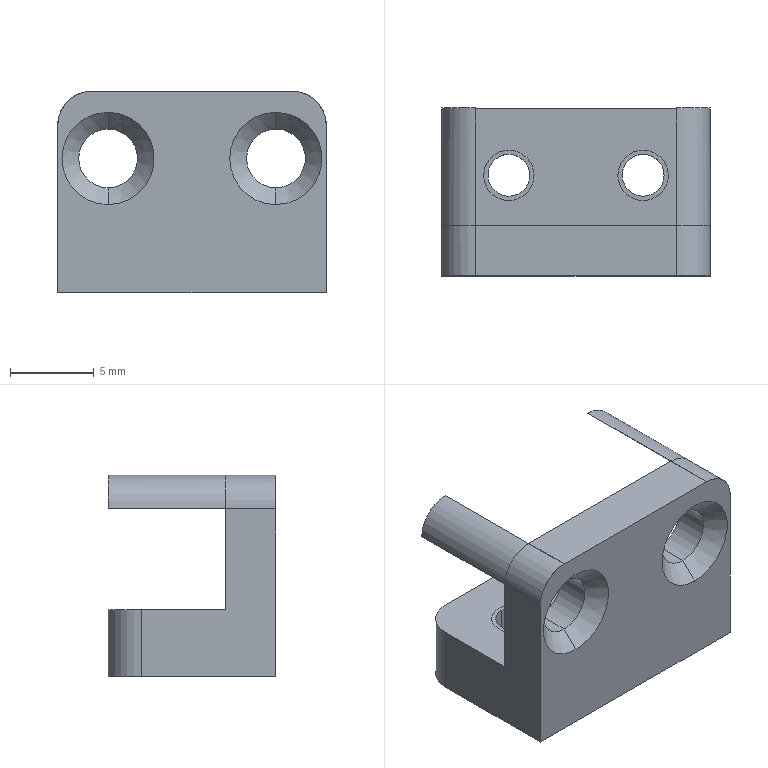CAM job | Mastercam | mm | 12 operations | part box 16 x 10 x 12
1. Facing | 8 - 8 平铣刀
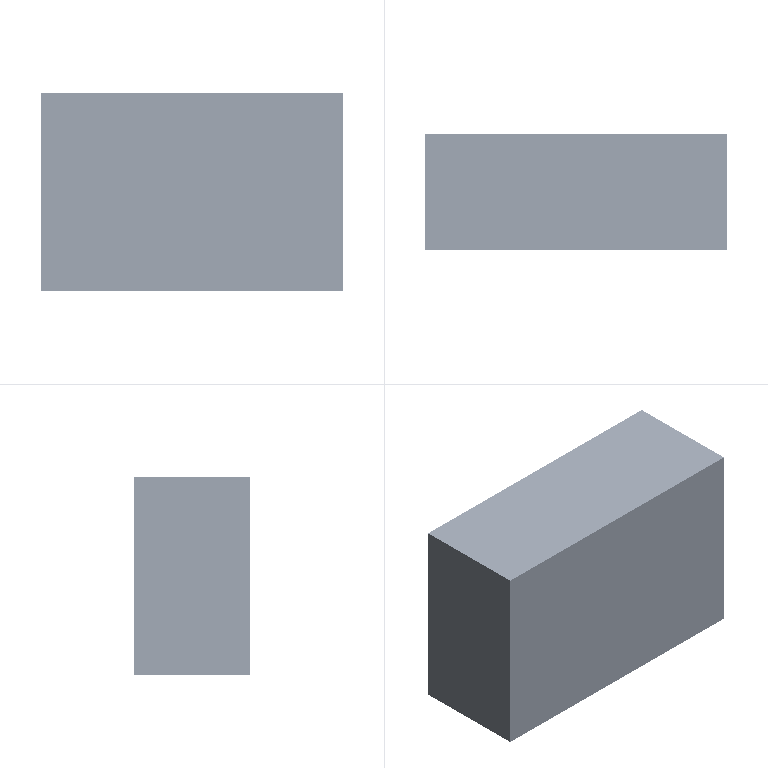2. Contour (Ramp) | 8 - 8 平铣刀
3. Contour (2D) | 8 - 8 平铣刀
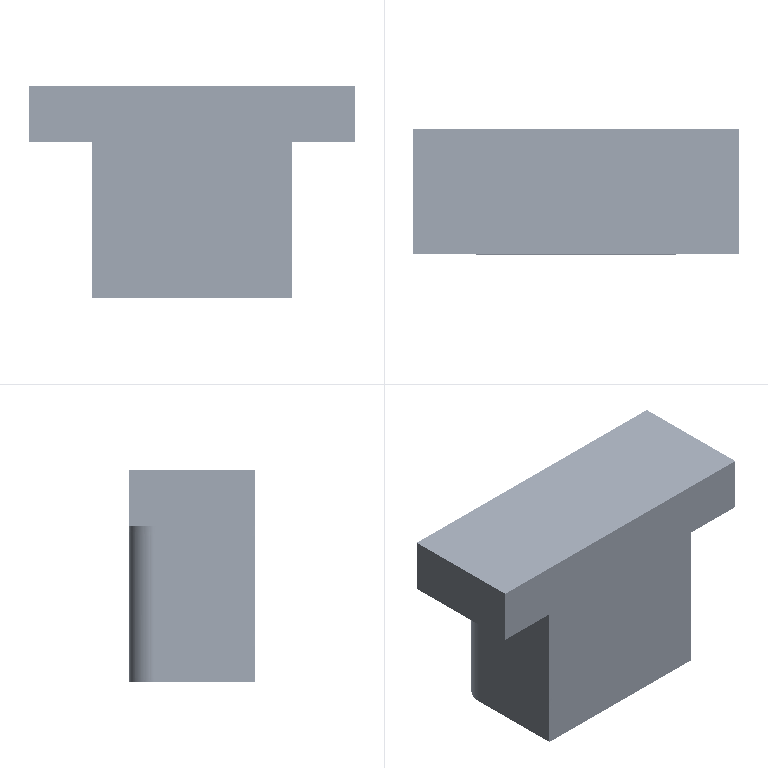4. Contour (2D chamfer) | 7 - 4 倒角刀
5. Drill/Counterbore | 7 - 4 倒角刀
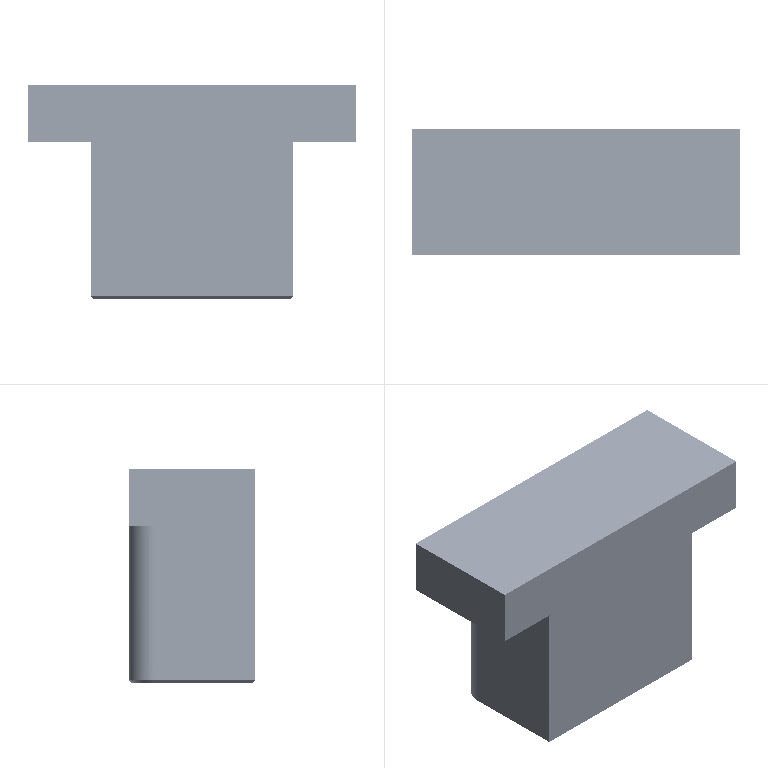6. Facing | 8 - 8 平铣刀
7. Surface Finish Flowline | 5 - 4 圆鼻铣刀
8. Contour (2D chamfer) | 7 - 4 倒角刀
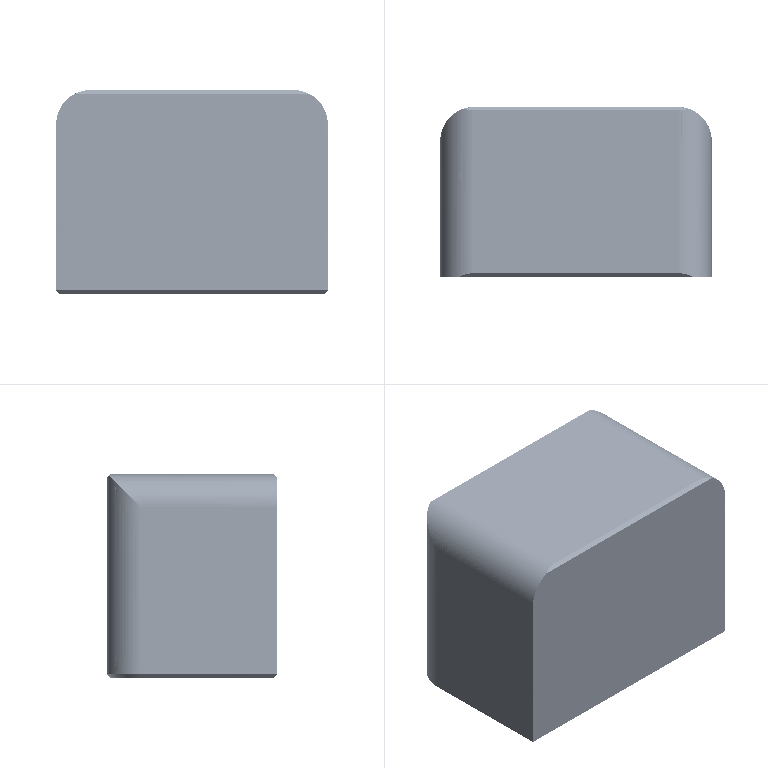9. Contour (Ramp) | 8 - 8 平铣刀
10. Contour (2D) | 8 - 8 平铣刀
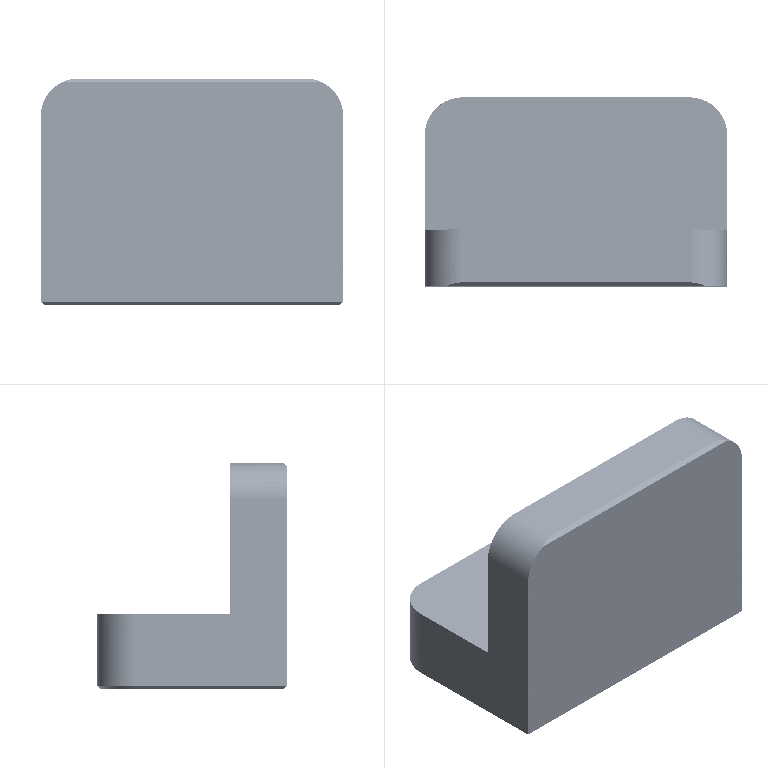11. Drill/Counterbore | 7 - 4 倒角刀
12. Contour (2D chamfer) | 7 - 4 倒角刀